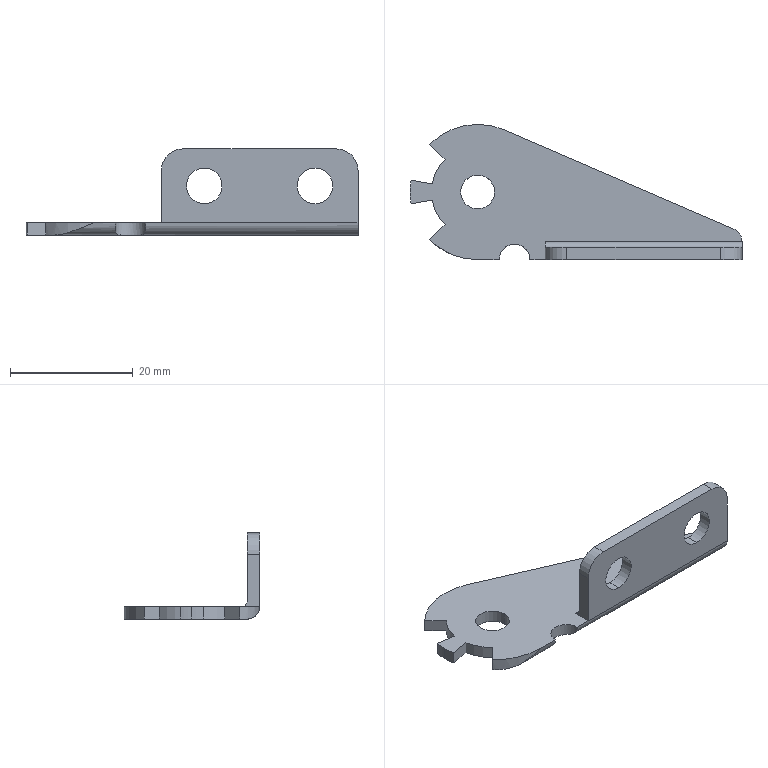Component | SolidWorks | MHPUS204-38-33-A-1_36-1 | 1 solid | 31 faces | box 54 x 22 x 14 mm | volume 2031 mm3 | cylinder 19 | plane 12 | commonest cylinder face diameters 22 x4 5.8 x4 5.5 x2 4 x2 15 x2 7 x2 5 x1 4.4 x1
STEP:
#1=COLOUR_RGB('',0.7922,0.8196,0.9333);
#2=FILL_AREA_STYLE_COLOUR('',#1);
#3=FILL_AREA_STYLE('',(#2));
#4=SURFACE_STYLE_FILL_AREA(#3);
#5=SURFACE_SIDE_STYLE('',(#4));
#6=SURFACE_STYLE_USAGE(.BOTH.,#5);
#7=PRESENTATION_STYLE_ASSIGNMENT((#6));
#8=CARTESIAN_POINT('',(0.1718,-3.898,2.047));
#9=VERTEX_POINT('',#8);
#10=CARTESIAN_POINT('',(-0.04475,-3.898,2.047));
#11=VERTEX_POINT('',#10);
#12=CARTESIAN_POINT('',(0.06352,-3.898,2.047));
#13=DIRECTION('',(0.,0.,-1.));
#14=DIRECTION('',(-1.,0.,0.));
#15=AXIS2_PLACEMENT_3D('',#12,#13,#14);
#16=CIRCLE('',#15,0.1083);
#17=EDGE_CURVE('',#9,#11,#16,.T.);
#18=ORIENTED_EDGE('',*,*,#17,.F.);
#19=CARTESIAN_POINT('',(0.1718,-3.898,1.969));
#20=VERTEX_POINT('',#19);
#21=CARTESIAN_POINT('',(0.1718,-3.898,1.969));
#22=DIRECTION('',(0.,0.,-1.));
#23=VECTOR('',#22,39.37);
#24=LINE('',#21,#23);
#25=EDGE_CURVE('',#9,#20,#24,.T.);
#26=ORIENTED_EDGE('',*,*,#25,.T.);
#27=CARTESIAN_POINT('',(-0.04475,-3.898,1.969));
#28=VERTEX_POINT('',#27);
#29=CARTESIAN_POINT('',(0.06352,-3.898,1.969));
#30=DIRECTION('',(0.,0.,-1.));
#31=DIRECTION('',(-1.,0.,0.));
#32=AXIS2_PLACEMENT_3D('',#29,#30,#31);
#33=CIRCLE('',#32,0.1083);
#34=EDGE_CURVE('',#20,#28,#33,.T.);
#35=ORIENTED_EDGE('',*,*,#34,.T.);
#36=CARTESIAN_POINT('',(-0.04475,-3.898,1.969));
#37=DIRECTION('',(0.,0.,-1.));
#38=VECTOR('',#37,39.37);
#39=LINE('',#36,#38);
#40=EDGE_CURVE('',#11,#28,#39,.T.);
#41=ORIENTED_EDGE('',*,*,#40,.F.);
#42=EDGE_LOOP('',(#18,#26,#35,#41));
#43=FACE_OUTER_BOUND('',#42,.T.);
#44=CARTESIAN_POINT('',(0.06352,-3.898,1.969));
#45=DIRECTION('',(0.,0.,-1.));
#46=DIRECTION('',(-1.,0.,0.));
#47=AXIS2_PLACEMENT_3D('',#44,#45,#46);
#48=CYLINDRICAL_SURFACE('',#47,0.1083);
#49=ADVANCED_FACE('',(#43),#48,.F.);
#50=CARTESIAN_POINT('',(-0.363,-3.973,2.047));
#51=VERTEX_POINT('',#50);
#52=CARTESIAN_POINT('',(-0.3696,-3.898,2.047));
#53=VERTEX_POINT('',#52);
#54=CARTESIAN_POINT('',(0.06352,-3.898,2.047));
#55=DIRECTION('',(0.,0.,-1.));
#56=DIRECTION('',(-1.,0.,0.));
#57=AXIS2_PLACEMENT_3D('',#54,#55,#56);
#58=CIRCLE('',#57,0.4331);
#59=EDGE_CURVE('',#51,#53,#58,.T.);
#60=ORIENTED_EDGE('',*,*,#59,.T.);
#61=CARTESIAN_POINT('',(-0.3696,-3.898,1.969));
#62=VERTEX_POINT('',#61);
#63=CARTESIAN_POINT('',(-0.3696,-3.898,1.969));
#64=DIRECTION('',(0.,0.,-1.));
#65=VECTOR('',#64,39.37);
#66=LINE('',#63,#65);
#67=EDGE_CURVE('',#53,#62,#66,.T.);
#68=ORIENTED_EDGE('',*,*,#67,.T.);
#69=CARTESIAN_POINT('',(-0.363,-3.973,1.969));
#70=VERTEX_POINT('',#69);
#71=CARTESIAN_POINT('',(0.06352,-3.898,1.969));
#72=DIRECTION('',(0.,0.,1.));
#73=DIRECTION('',(-1.,0.,0.));
#74=AXIS2_PLACEMENT_3D('',#71,#72,#73);
#75=CIRCLE('',#74,0.4331);
#76=EDGE_CURVE('',#62,#70,#75,.T.);
#77=ORIENTED_EDGE('',*,*,#76,.T.);
#78=CARTESIAN_POINT('',(-0.363,-3.973,1.969));
#79=DIRECTION('',(0.,0.,-1.));
#80=VECTOR('',#79,39.37);
#81=LINE('',#78,#80);
#82=EDGE_CURVE('',#51,#70,#81,.T.);
#83=ORIENTED_EDGE('',*,*,#82,.F.);
#84=EDGE_LOOP('',(#60,#68,#77,#83));
#85=FACE_OUTER_BOUND('',#84,.T.);
#86=CARTESIAN_POINT('',(0.06352,-3.898,1.969));
#87=DIRECTION('',(0.,0.,-1.));
#88=DIRECTION('',(-1.,0.,0.));
#89=AXIS2_PLACEMENT_3D('',#86,#87,#88);
#90=CYLINDRICAL_SURFACE('',#89,0.4331);
#91=ADVANCED_FACE('',(#85),#90,.T.);
#92=CARTESIAN_POINT('',(0.7722,-4.252,2.169));
#93=VERTEX_POINT('',#92);
#94=CARTESIAN_POINT('',(0.7722,-4.252,2.398));
#95=VERTEX_POINT('',#94);
#96=CARTESIAN_POINT('',(0.7722,-4.252,2.283));
#97=DIRECTION('',(0.,1.,0.));
#98=DIRECTION('',(0.,0.,-1.));
#99=AXIS2_PLACEMENT_3D('',#96,#97,#98);
#100=CIRCLE('',#99,0.1142);
#101=EDGE_CURVE('',#93,#95,#100,.T.);
#102=ORIENTED_EDGE('',*,*,#101,.T.);
#103=CARTESIAN_POINT('',(0.7722,-4.331,2.398));
#104=VERTEX_POINT('',#103);
#105=CARTESIAN_POINT('',(0.7722,-4.331,2.398));
#106=DIRECTION('',(0.,-1.,0.));
#107=VECTOR('',#106,39.37);
#108=LINE('',#105,#107);
#109=EDGE_CURVE('',#95,#104,#108,.T.);
#110=ORIENTED_EDGE('',*,*,#109,.T.);
#111=CARTESIAN_POINT('',(0.7722,-4.331,2.169));
#112=VERTEX_POINT('',#111);
#113=CARTESIAN_POINT('',(0.7722,-4.331,2.283));
#114=DIRECTION('',(0.,1.,0.));
#115=DIRECTION('',(0.,0.,-1.));
#116=AXIS2_PLACEMENT_3D('',#113,#114,#115);
#117=CIRCLE('',#116,0.1142);
#118=EDGE_CURVE('',#112,#104,#117,.T.);
#119=ORIENTED_EDGE('',*,*,#118,.F.);
#120=CARTESIAN_POINT('',(0.7722,-4.331,2.169));
#121=DIRECTION('',(0.,-1.,0.));
#122=VECTOR('',#121,39.37);
#123=LINE('',#120,#122);
#124=EDGE_CURVE('',#93,#112,#123,.T.);
#125=ORIENTED_EDGE('',*,*,#124,.F.);
#126=EDGE_LOOP('',(#102,#110,#119,#125));
#127=FACE_OUTER_BOUND('',#126,.T.);
#128=CARTESIAN_POINT('',(0.7722,-4.331,2.283));
#129=DIRECTION('',(0.,-1.,0.));
#130=DIRECTION('',(0.,0.,-1.));
#131=AXIS2_PLACEMENT_3D('',#128,#129,#130);
#132=CYLINDRICAL_SURFACE('',#131,0.1142);
#133=ADVANCED_FACE('',(#127),#132,.F.);
#134=CARTESIAN_POINT('',(1.481,-4.252,2.169));
#135=VERTEX_POINT('',#134);
#136=CARTESIAN_POINT('',(1.481,-4.252,2.398));
#137=VERTEX_POINT('',#136);
#138=CARTESIAN_POINT('',(1.481,-4.252,2.283));
#139=DIRECTION('',(0.,1.,0.));
#140=DIRECTION('',(0.,0.,-1.));
#141=AXIS2_PLACEMENT_3D('',#138,#139,#140);
#142=CIRCLE('',#141,0.1142);
#143=EDGE_CURVE('',#135,#137,#142,.T.);
#144=ORIENTED_EDGE('',*,*,#143,.T.);
#145=CARTESIAN_POINT('',(1.481,-4.331,2.398));
#146=VERTEX_POINT('',#145);
#147=CARTESIAN_POINT('',(1.481,-4.331,2.398));
#148=DIRECTION('',(0.,-1.,0.));
#149=VECTOR('',#148,39.37);
#150=LINE('',#147,#149);
#151=EDGE_CURVE('',#137,#146,#150,.T.);
#152=ORIENTED_EDGE('',*,*,#151,.T.);
#153=CARTESIAN_POINT('',(1.481,-4.331,2.169));
#154=VERTEX_POINT('',#153);
#155=CARTESIAN_POINT('',(1.481,-4.331,2.283));
#156=DIRECTION('',(0.,1.,0.));
#157=DIRECTION('',(0.,0.,-1.));
#158=AXIS2_PLACEMENT_3D('',#155,#156,#157);
#159=CIRCLE('',#158,0.1142);
#160=EDGE_CURVE('',#154,#146,#159,.T.);
#161=ORIENTED_EDGE('',*,*,#160,.F.);
#162=CARTESIAN_POINT('',(1.481,-4.331,2.169));
#163=DIRECTION('',(0.,-1.,0.));
#164=VECTOR('',#163,39.37);
#165=LINE('',#162,#164);
#166=EDGE_CURVE('',#135,#154,#165,.T.);
#167=ORIENTED_EDGE('',*,*,#166,.F.);
#168=EDGE_LOOP('',(#144,#152,#161,#167));
#169=FACE_OUTER_BOUND('',#168,.T.);
#170=CARTESIAN_POINT('',(1.481,-4.331,2.283));
#171=DIRECTION('',(0.,-1.,0.));
#172=DIRECTION('',(0.,0.,-1.));
#173=AXIS2_PLACEMENT_3D('',#170,#171,#172);
#174=CYLINDRICAL_SURFACE('',#173,0.1142);
#175=ADVANCED_FACE('',(#169),#174,.F.);
#176=CARTESIAN_POINT('',(0.06352,-3.898,1.969));
#177=DIRECTION('',(0.,0.,-1.));
#178=DIRECTION('',(-1.,0.,0.));
#179=AXIS2_PLACEMENT_3D('',#176,#177,#178);
#180=CIRCLE('',#179,0.1083);
#181=EDGE_CURVE('',#28,#20,#180,.T.);
#182=ORIENTED_EDGE('',*,*,#181,.F.);
#183=ORIENTED_EDGE('',*,*,#34,.F.);
#184=EDGE_LOOP('',(#182,#183));
#185=FACE_BOUND('',#184,.T.);
#186=CARTESIAN_POINT('',(-0.1855,-4.252,1.969));
#187=VERTEX_POINT('',#186);
#188=CARTESIAN_POINT('',(0.2407,-4.252,1.969));
#189=VERTEX_POINT('',#188);
#190=CARTESIAN_POINT('',(0.06352,-4.252,1.969));
#191=DIRECTION('',(1.,0.,0.));
#192=VECTOR('',#191,39.37);
#193=LINE('',#190,#192);
#194=EDGE_CURVE('',#187,#189,#193,.T.);
#195=ORIENTED_EDGE('',*,*,#194,.F.);
#196=CARTESIAN_POINT('',(-0.2427,-4.204,1.969));
#197=VERTEX_POINT('',#196);
#198=CARTESIAN_POINT('',(0.06352,-3.898,1.969));
#199=DIRECTION('',(0.,0.,1.));
#200=DIRECTION('',(-1.,-0.,0.));
#201=AXIS2_PLACEMENT_3D('',#198,#199,#200);
#202=CIRCLE('',#201,0.4331);
#203=EDGE_CURVE('',#197,#187,#202,.T.);
#204=ORIENTED_EDGE('',*,*,#203,.F.);
#205=CARTESIAN_POINT('',(-0.1453,-4.106,1.969));
#206=VERTEX_POINT('',#205);
#207=CARTESIAN_POINT('',(-0.1453,-4.106,1.969));
#208=DIRECTION('',(-0.7071,-0.7071,0.));
#209=VECTOR('',#208,39.37);
#210=LINE('',#207,#209);
#211=EDGE_CURVE('',#206,#197,#210,.T.);
#212=ORIENTED_EDGE('',*,*,#211,.F.);
#213=CARTESIAN_POINT('',(-0.2273,-3.949,1.969));
#214=VERTEX_POINT('',#213);
#215=CARTESIAN_POINT('',(0.06352,-3.898,1.969));
#216=DIRECTION('',(0.,0.,1.));
#217=DIRECTION('',(-1.,0.,0.));
#218=AXIS2_PLACEMENT_3D('',#215,#216,#217);
#219=CIRCLE('',#218,0.2953);
#220=EDGE_CURVE('',#214,#206,#219,.T.);
#221=ORIENTED_EDGE('',*,*,#220,.F.);
#222=CARTESIAN_POINT('',(-0.363,-3.973,1.969));
#223=DIRECTION('',(0.9848,0.1736,0.));
#224=VECTOR('',#223,39.37);
#225=LINE('',#222,#224);
#226=EDGE_CURVE('',#70,#214,#225,.T.);
#227=ORIENTED_EDGE('',*,*,#226,.F.);
#228=ORIENTED_EDGE('',*,*,#76,.F.);
#229=CARTESIAN_POINT('',(-0.363,-3.822,1.969));
#230=VERTEX_POINT('',#229);
#231=CARTESIAN_POINT('',(0.06352,-3.898,1.969));
#232=DIRECTION('',(0.,0.,1.));
#233=DIRECTION('',(-1.,0.,0.));
#234=AXIS2_PLACEMENT_3D('',#231,#232,#233);
#235=CIRCLE('',#234,0.4331);
#236=EDGE_CURVE('',#230,#62,#235,.T.);
#237=ORIENTED_EDGE('',*,*,#236,.F.);
#238=CARTESIAN_POINT('',(-0.2273,-3.846,1.969));
#239=VERTEX_POINT('',#238);
#240=CARTESIAN_POINT('',(-0.2273,-3.846,1.969));
#241=DIRECTION('',(-0.9848,0.1736,0.));
#242=VECTOR('',#241,39.37);
#243=LINE('',#240,#242);
#244=EDGE_CURVE('',#239,#230,#243,.T.);
#245=ORIENTED_EDGE('',*,*,#244,.F.);
#246=CARTESIAN_POINT('',(-0.1453,-3.689,1.969));
#247=VERTEX_POINT('',#246);
#248=CARTESIAN_POINT('',(0.06352,-3.898,1.969));
#249=DIRECTION('',(0.,0.,1.));
#250=DIRECTION('',(-1.,0.,0.));
#251=AXIS2_PLACEMENT_3D('',#248,#249,#250);
#252=CIRCLE('',#251,0.2953);
#253=EDGE_CURVE('',#247,#239,#252,.T.);
#254=ORIENTED_EDGE('',*,*,#253,.F.);
#255=CARTESIAN_POINT('',(-0.2427,-3.591,1.969));
#256=VERTEX_POINT('',#255);
#257=CARTESIAN_POINT('',(-0.2427,-3.591,1.969));
#258=DIRECTION('',(0.7071,-0.7071,0.));
#259=VECTOR('',#258,39.37);
#260=LINE('',#257,#259);
#261=EDGE_CURVE('',#256,#247,#260,.T.);
#262=ORIENTED_EDGE('',*,*,#261,.F.);
#263=CARTESIAN_POINT('',(0.2353,-3.5,1.969));
#264=VERTEX_POINT('',#263);
#265=CARTESIAN_POINT('',(0.06352,-3.898,1.969));
#266=DIRECTION('',(0.,0.,1.));
#267=DIRECTION('',(-1.,-0.,0.));
#268=AXIS2_PLACEMENT_3D('',#265,#266,#267);
#269=CIRCLE('',#268,0.4331);
#270=EDGE_CURVE('',#264,#256,#269,.T.);
#271=ORIENTED_EDGE('',*,*,#270,.F.);
#272=CARTESIAN_POINT('',(1.704,-4.135,1.969));
#273=VERTEX_POINT('',#272);
#274=CARTESIAN_POINT('',(1.704,-4.135,1.969));
#275=DIRECTION('',(-0.9179,0.3967,0.));
#276=VECTOR('',#275,39.37);
#277=LINE('',#274,#276);
#278=EDGE_CURVE('',#273,#264,#277,.T.);
#279=ORIENTED_EDGE('',*,*,#278,.F.);
#280=CARTESIAN_POINT('',(1.756,-4.214,1.969));
#281=VERTEX_POINT('',#280);
#282=CARTESIAN_POINT('',(1.67,-4.214,1.969));
#283=DIRECTION('',(0.,0.,1.));
#284=DIRECTION('',(-1.,-0.,0.));
#285=AXIS2_PLACEMENT_3D('',#282,#283,#284);
#286=CIRCLE('',#285,0.08661);
#287=EDGE_CURVE('',#281,#273,#286,.T.);
#288=ORIENTED_EDGE('',*,*,#287,.F.);
#289=CARTESIAN_POINT('',(1.756,-4.252,1.969));
#290=VERTEX_POINT('',#289);
#291=CARTESIAN_POINT('',(1.756,-4.214,1.969));
#292=DIRECTION('',(0.,1.,0.));
#293=VECTOR('',#292,39.37);
#294=LINE('',#291,#293);
#295=EDGE_CURVE('',#290,#281,#294,.T.);
#296=ORIENTED_EDGE('',*,*,#295,.F.);
#297=CARTESIAN_POINT('',(0.3588,-4.252,1.969));
#298=VERTEX_POINT('',#297);
#299=CARTESIAN_POINT('',(0.06352,-4.252,1.969));
#300=DIRECTION('',(1.,0.,0.));
#301=VECTOR('',#300,39.37);
#302=LINE('',#299,#301);
#303=EDGE_CURVE('',#298,#290,#302,.T.);
#304=ORIENTED_EDGE('',*,*,#303,.F.);
#305=CARTESIAN_POINT('',(0.2997,-4.331,1.969));
#306=DIRECTION('',(0.,0.,-1.));
#307=DIRECTION('',(-1.,0.,0.));
#308=AXIS2_PLACEMENT_3D('',#305,#306,#307);
#309=CIRCLE('',#308,0.09843);
#310=EDGE_CURVE('',#189,#298,#309,.T.);
#311=ORIENTED_EDGE('',*,*,#310,.F.);
#312=EDGE_LOOP('',(#195,#204,#212,#221,#227,#228,#237,#245,#254,#262,#271,#279,#288,#296,#304,#311));
#313=FACE_OUTER_BOUND('',#312,.T.);
#314=CARTESIAN_POINT('',(0.06352,-4.331,1.969));
#315=DIRECTION('',(0.,0.,1.));
#316=DIRECTION('',(1.,0.,0.));
#317=AXIS2_PLACEMENT_3D('',#314,#315,#316);
#318=PLANE('',#317);
#319=ADVANCED_FACE('',(#185,#313),#318,.F.);
#320=ORIENTED_EDGE('',*,*,#25,.F.);
#321=CARTESIAN_POINT('',(0.06352,-3.898,2.047));
#322=DIRECTION('',(0.,0.,-1.));
#323=DIRECTION('',(-1.,0.,0.));
#324=AXIS2_PLACEMENT_3D('',#321,#322,#323);
#325=CIRCLE('',#324,0.1083);
#326=EDGE_CURVE('',#11,#9,#325,.T.);
#327=ORIENTED_EDGE('',*,*,#326,.F.);
#328=ORIENTED_EDGE('',*,*,#40,.T.);
#329=ORIENTED_EDGE('',*,*,#181,.T.);
#330=EDGE_LOOP('',(#320,#327,#328,#329));
#331=FACE_OUTER_BOUND('',#330,.T.);
#332=CARTESIAN_POINT('',(0.06352,-3.898,1.969));
#333=DIRECTION('',(0.,0.,-1.));
#334=DIRECTION('',(-1.,0.,0.));
#335=AXIS2_PLACEMENT_3D('',#332,#333,#334);
#336=CYLINDRICAL_SURFACE('',#335,0.1083);
#337=ADVANCED_FACE('',(#331),#336,.F.);
#338=CARTESIAN_POINT('',(0.2013,-4.331,2.047));
#339=VERTEX_POINT('',#338);
#340=CARTESIAN_POINT('',(0.3982,-4.331,2.047));
#341=VERTEX_POINT('',#340);
#342=CARTESIAN_POINT('',(0.2997,-4.331,2.047));
#343=DIRECTION('',(0.,0.,-1.));
#344=DIRECTION('',(-1.,0.,0.));
#345=AXIS2_PLACEMENT_3D('',#342,#343,#344);
#346=CIRCLE('',#345,0.09843);
#347=EDGE_CURVE('',#339,#341,#346,.T.);
#348=ORIENTED_EDGE('',*,*,#347,.F.);
#349=CARTESIAN_POINT('',(0.2407,-4.252,1.969));
#350=CARTESIAN_POINT('',(0.2361,-4.255,1.969));
#351=CARTESIAN_POINT('',(0.2319,-4.259,1.969));
#352=CARTESIAN_POINT('',(0.2243,-4.267,1.97));
#353=CARTESIAN_POINT('',(0.2207,-4.272,1.971));
#354=CARTESIAN_POINT('',(0.2147,-4.281,1.974));
#355=CARTESIAN_POINT('',(0.2122,-4.285,1.976));
#356=CARTESIAN_POINT('',(0.208,-4.295,1.981));
#357=CARTESIAN_POINT('',(0.2064,-4.299,1.984));
#358=CARTESIAN_POINT('',(0.204,-4.307,1.991));
#359=CARTESIAN_POINT('',(0.2032,-4.311,1.995));
#360=CARTESIAN_POINT('',(0.2021,-4.318,2.004));
#361=CARTESIAN_POINT('',(0.2018,-4.321,2.009));
#362=CARTESIAN_POINT('',(0.2014,-4.326,2.019));
#363=CARTESIAN_POINT('',(0.2014,-4.328,2.025));
#364=CARTESIAN_POINT('',(0.2013,-4.33,2.036));
#365=CARTESIAN_POINT('',(0.2013,-4.331,2.042));
#366=CARTESIAN_POINT('',(0.2013,-4.331,2.047));
#367=B_SPLINE_CURVE_WITH_KNOTS('',3,(#349,#350,#351,#352,#353,#354,#355,#356,#357,#358,#359,#360,#361,#362,#363,#364,#365,#366),.UNSPECIFIED.,.F.,.F.,(4,2,2,2,2,2,2,2,4),(0.,0.0004287,0.0008574,0.001286,0.001715,0.002144,0.002572,0.003001,0.00343),.UNSPECIFIED.);
#368=EDGE_CURVE('',#189,#339,#367,.T.);
#369=ORIENTED_EDGE('',*,*,#368,.F.);
#370=ORIENTED_EDGE('',*,*,#310,.T.);
#371=CARTESIAN_POINT('',(0.3982,-4.331,2.047));
#372=CARTESIAN_POINT('',(0.3982,-4.331,2.042));
#373=CARTESIAN_POINT('',(0.3982,-4.33,2.036));
#374=CARTESIAN_POINT('',(0.3981,-4.328,2.025));
#375=CARTESIAN_POINT('',(0.3981,-4.326,2.019));
#376=CARTESIAN_POINT('',(0.3977,-4.321,2.009));
#377=CARTESIAN_POINT('',(0.3974,-4.318,2.004));
#378=CARTESIAN_POINT('',(0.3963,-4.311,1.995));
#379=CARTESIAN_POINT('',(0.3955,-4.308,1.991));
#380=CARTESIAN_POINT('',(0.3931,-4.299,1.984));
#381=CARTESIAN_POINT('',(0.3915,-4.295,1.981));
#382=CARTESIAN_POINT('',(0.3874,-4.286,1.976));
#383=CARTESIAN_POINT('',(0.3849,-4.281,1.974));
#384=CARTESIAN_POINT('',(0.3757,-4.267,1.969));
#385=CARTESIAN_POINT('',(0.3679,-4.259,1.969));
#386=CARTESIAN_POINT('',(0.3588,-4.252,1.969));
#387=B_SPLINE_CURVE_WITH_KNOTS('',3,(#371,#372,#373,#374,#375,#376,#377,#378,#379,#380,#381,#382,#383,#384,#385,#386),.UNSPECIFIED.,.F.,.F.,(4,2,2,2,2,2,2,4),(0.,0.0004284,0.0008569,0.001285,0.001714,0.002142,0.002571,0.003428),.UNSPECIFIED.);
#388=EDGE_CURVE('',#341,#298,#387,.T.);
#389=ORIENTED_EDGE('',*,*,#388,.F.);
#390=EDGE_LOOP('',(#348,#369,#370,#389));
#391=FACE_OUTER_BOUND('',#390,.T.);
#392=CARTESIAN_POINT('',(0.2997,-4.331,1.969));
#393=DIRECTION('',(0.,0.,-1.));
#394=DIRECTION('',(-1.,0.,0.));
#395=AXIS2_PLACEMENT_3D('',#392,#393,#394);
#396=CYLINDRICAL_SURFACE('',#395,0.09843);
#397=ADVANCED_FACE('',(#391),#396,.F.);
#398=CARTESIAN_POINT('',(0.06352,-4.331,2.047));
#399=VERTEX_POINT('',#398);
#400=CARTESIAN_POINT('',(0.06352,-4.331,2.047));
#401=CARTESIAN_POINT('',(0.04212,-4.331,2.038));
#402=CARTESIAN_POINT('',(0.02068,-4.329,2.029));
#403=CARTESIAN_POINT('',(-0.02198,-4.323,2.011));
#404=CARTESIAN_POINT('',(-0.04301,-4.318,2.003));
#405=CARTESIAN_POINT('',(-0.0743,-4.308,1.992));
#406=CARTESIAN_POINT('',(-0.08469,-4.305,1.989));
#407=CARTESIAN_POINT('',(-0.1054,-4.297,1.982));
#408=CARTESIAN_POINT('',(-0.1158,-4.292,1.979));
#409=CARTESIAN_POINT('',(-0.1465,-4.277,1.972));
#410=CARTESIAN_POINT('',(-0.1663,-4.265,1.969));
#411=CARTESIAN_POINT('',(-0.1855,-4.252,1.969));
#412=B_SPLINE_CURVE_WITH_KNOTS('',3,(#400,#401,#402,#403,#404,#405,#406,#407,#408,#409,#410,#411),.UNSPECIFIED.,.F.,.F.,(4,2,2,2,2,4),(-0.00002098,0.001752,0.003524,0.004411,0.005297,0.00707),.UNSPECIFIED.);
#413=EDGE_CURVE('',#399,#187,#412,.T.);
#414=ORIENTED_EDGE('',*,*,#413,.T.);
#415=ORIENTED_EDGE('',*,*,#194,.T.);
#416=ORIENTED_EDGE('',*,*,#368,.T.);
#417=CARTESIAN_POINT('',(1.756,-4.331,2.047));
#418=DIRECTION('',(-1.,0.,0.));
#419=VECTOR('',#418,39.37);
#420=LINE('',#417,#419);
#421=EDGE_CURVE('',#339,#399,#420,.T.);
#422=ORIENTED_EDGE('',*,*,#421,.T.);
#423=EDGE_LOOP('',(#414,#415,#416,#422));
#424=FACE_OUTER_BOUND('',#423,.T.);
#425=CARTESIAN_POINT('',(1.756,-4.252,2.047));
#426=DIRECTION('',(1.,0.,0.));
#427=DIRECTION('',(0.,0.,-1.));
#428=AXIS2_PLACEMENT_3D('',#425,#426,#427);
#429=CYLINDRICAL_SURFACE('',#428,0.07874);
#430=ADVANCED_FACE('',(#424),#429,.T.);
#431=ORIENTED_EDGE('',*,*,#203,.T.);
#432=ORIENTED_EDGE('',*,*,#413,.F.);
#433=CARTESIAN_POINT('',(-0.2427,-4.204,2.047));
#434=VERTEX_POINT('',#433);
#435=CARTESIAN_POINT('',(0.06352,-3.898,2.047));
#436=DIRECTION('',(0.,0.,-1.));
#437=DIRECTION('',(-1.,0.,0.));
#438=AXIS2_PLACEMENT_3D('',#435,#436,#437);
#439=CIRCLE('',#438,0.4331);
#440=EDGE_CURVE('',#399,#434,#439,.T.);
#441=ORIENTED_EDGE('',*,*,#440,.T.);
#442=CARTESIAN_POINT('',(-0.2427,-4.204,1.969));
#443=DIRECTION('',(0.,0.,-1.));
#444=VECTOR('',#443,39.37);
#445=LINE('',#442,#444);
#446=EDGE_CURVE('',#434,#197,#445,.T.);
#447=ORIENTED_EDGE('',*,*,#446,.T.);
#448=EDGE_LOOP('',(#431,#432,#441,#447));
#449=FACE_OUTER_BOUND('',#448,.T.);
#450=CARTESIAN_POINT('',(0.06352,-3.898,1.969));
#451=DIRECTION('',(0.,0.,-1.));
#452=DIRECTION('',(-1.,0.,0.));
#453=AXIS2_PLACEMENT_3D('',#450,#451,#452);
#454=CYLINDRICAL_SURFACE('',#453,0.4331);
#455=ADVANCED_FACE('',(#449),#454,.T.);
#456=ORIENTED_EDGE('',*,*,#211,.T.);
#457=ORIENTED_EDGE('',*,*,#446,.F.);
#458=CARTESIAN_POINT('',(-0.1453,-4.106,2.047));
#459=VERTEX_POINT('',#458);
#460=CARTESIAN_POINT('',(-0.2427,-4.204,2.047));
#461=DIRECTION('',(0.7071,0.7071,0.));
#462=VECTOR('',#461,39.37);
#463=LINE('',#460,#462);
#464=EDGE_CURVE('',#434,#459,#463,.T.);
#465=ORIENTED_EDGE('',*,*,#464,.T.);
#466=CARTESIAN_POINT('',(-0.1453,-4.106,1.969));
#467=DIRECTION('',(0.,0.,-1.));
#468=VECTOR('',#467,39.37);
#469=LINE('',#466,#468);
#470=EDGE_CURVE('',#459,#206,#469,.T.);
#471=ORIENTED_EDGE('',*,*,#470,.T.);
#472=EDGE_LOOP('',(#456,#457,#465,#471));
#473=FACE_OUTER_BOUND('',#472,.T.);
#474=CARTESIAN_POINT('',(-0.2427,-4.204,1.969));
#475=DIRECTION('',(-0.7071,0.7071,0.));
#476=DIRECTION('',(-0.7071,-0.7071,0.));
#477=AXIS2_PLACEMENT_3D('',#474,#475,#476);
#478=PLANE('',#477);
#479=ADVANCED_FACE('',(#473),#478,.T.);
#480=ORIENTED_EDGE('',*,*,#220,.T.);
#481=ORIENTED_EDGE('',*,*,#470,.F.);
#482=CARTESIAN_POINT('',(-0.2273,-3.949,2.047));
#483=VERTEX_POINT('',#482);
#484=CARTESIAN_POINT('',(0.06352,-3.898,2.047));
#485=DIRECTION('',(0.,0.,-1.));
#486=DIRECTION('',(-1.,0.,0.));
#487=AXIS2_PLACEMENT_3D('',#484,#485,#486);
#488=CIRCLE('',#487,0.2953);
#489=EDGE_CURVE('',#459,#483,#488,.T.);
#490=ORIENTED_EDGE('',*,*,#489,.T.);
#491=CARTESIAN_POINT('',(-0.2273,-3.949,1.969));
#492=DIRECTION('',(0.,0.,-1.));
#493=VECTOR('',#492,39.37);
#494=LINE('',#491,#493);
#495=EDGE_CURVE('',#483,#214,#494,.T.);
#496=ORIENTED_EDGE('',*,*,#495,.T.);
#497=EDGE_LOOP('',(#480,#481,#490,#496));
#498=FACE_OUTER_BOUND('',#497,.T.);
#499=CARTESIAN_POINT('',(0.06352,-3.898,1.969));
#500=DIRECTION('',(0.,0.,-1.));
#501=DIRECTION('',(-1.,0.,0.));
#502=AXIS2_PLACEMENT_3D('',#499,#500,#501);
#503=CYLINDRICAL_SURFACE('',#502,0.2953);
#504=ADVANCED_FACE('',(#498),#503,.T.);
#505=ORIENTED_EDGE('',*,*,#226,.T.);
#506=ORIENTED_EDGE('',*,*,#495,.F.);
#507=CARTESIAN_POINT('',(-0.2273,-3.949,2.047));
#508=DIRECTION('',(-0.9848,-0.1736,0.));
#509=VECTOR('',#508,39.37);
#510=LINE('',#507,#509);
#511=EDGE_CURVE('',#483,#51,#510,.T.);
#512=ORIENTED_EDGE('',*,*,#511,.T.);
#513=ORIENTED_EDGE('',*,*,#82,.T.);
#514=EDGE_LOOP('',(#505,#506,#512,#513));
#515=FACE_OUTER_BOUND('',#514,.T.);
#516=CARTESIAN_POINT('',(-0.2273,-3.949,1.969));
#517=DIRECTION('',(0.1736,-0.9848,0.));
#518=DIRECTION('',(0.9848,0.1736,0.));
#519=AXIS2_PLACEMENT_3D('',#516,#517,#518);
#520=PLANE('',#519);
#521=ADVANCED_FACE('',(#515),#520,.T.);
#522=ORIENTED_EDGE('',*,*,#67,.F.);
#523=CARTESIAN_POINT('',(-0.363,-3.822,2.047));
#524=VERTEX_POINT('',#523);
#525=CARTESIAN_POINT('',(0.06352,-3.898,2.047));
#526=DIRECTION('',(0.,0.,-1.));
#527=DIRECTION('',(-1.,0.,0.));
#528=AXIS2_PLACEMENT_3D('',#525,#526,#527);
#529=CIRCLE('',#528,0.4331);
#530=EDGE_CURVE('',#53,#524,#529,.T.);
#531=ORIENTED_EDGE('',*,*,#530,.T.);
#532=CARTESIAN_POINT('',(-0.363,-3.822,1.969));
#533=DIRECTION('',(0.,0.,-1.));
#534=VECTOR('',#533,39.37);
#535=LINE('',#532,#534);
#536=EDGE_CURVE('',#524,#230,#535,.T.);
#537=ORIENTED_EDGE('',*,*,#536,.T.);
#538=ORIENTED_EDGE('',*,*,#236,.T.);
#539=EDGE_LOOP('',(#522,#531,#537,#538));
#540=FACE_OUTER_BOUND('',#539,.T.);
#541=CARTESIAN_POINT('',(0.06352,-3.898,1.969));
#542=DIRECTION('',(0.,0.,-1.));
#543=DIRECTION('',(-1.,0.,0.));
#544=AXIS2_PLACEMENT_3D('',#541,#542,#543);
#545=CYLINDRICAL_SURFACE('',#544,0.4331);
#546=ADVANCED_FACE('',(#540),#545,.T.);
#547=ORIENTED_EDGE('',*,*,#244,.T.);
#548=ORIENTED_EDGE('',*,*,#536,.F.);
#549=CARTESIAN_POINT('',(-0.2273,-3.846,2.047));
#550=VERTEX_POINT('',#549);
#551=CARTESIAN_POINT('',(-0.363,-3.822,2.047));
#552=DIRECTION('',(0.9848,-0.1736,0.));
#553=VECTOR('',#552,39.37);
#554=LINE('',#551,#553);
#555=EDGE_CURVE('',#524,#550,#554,.T.);
#556=ORIENTED_EDGE('',*,*,#555,.T.);
#557=CARTESIAN_POINT('',(-0.2273,-3.846,1.969));
#558=DIRECTION('',(0.,0.,-1.));
#559=VECTOR('',#558,39.37);
#560=LINE('',#557,#559);
#561=EDGE_CURVE('',#550,#239,#560,.T.);
#562=ORIENTED_EDGE('',*,*,#561,.T.);
#563=EDGE_LOOP('',(#547,#548,#556,#562));
#564=FACE_OUTER_BOUND('',#563,.T.);
#565=CARTESIAN_POINT('',(-0.363,-3.822,1.969));
#566=DIRECTION('',(0.1736,0.9848,0.));
#567=DIRECTION('',(-0.9848,0.1736,0.));
#568=AXIS2_PLACEMENT_3D('',#565,#566,#567);
#569=PLANE('',#568);
#570=ADVANCED_FACE('',(#564),#569,.T.);
#571=ORIENTED_EDGE('',*,*,#253,.T.);
#572=ORIENTED_EDGE('',*,*,#561,.F.);
#573=CARTESIAN_POINT('',(-0.1453,-3.689,2.047));
#574=VERTEX_POINT('',#573);
#575=CARTESIAN_POINT('',(0.06352,-3.898,2.047));
#576=DIRECTION('',(0.,0.,-1.));
#577=DIRECTION('',(-1.,0.,0.));
#578=AXIS2_PLACEMENT_3D('',#575,#576,#577);
#579=CIRCLE('',#578,0.2953);
#580=EDGE_CURVE('',#550,#574,#579,.T.);
#581=ORIENTED_EDGE('',*,*,#580,.T.);
#582=CARTESIAN_POINT('',(-0.1453,-3.689,1.969));
#583=DIRECTION('',(0.,0.,-1.));
#584=VECTOR('',#583,39.37);
#585=LINE('',#582,#584);
#586=EDGE_CURVE('',#574,#247,#585,.T.);
#587=ORIENTED_EDGE('',*,*,#586,.T.);
#588=EDGE_LOOP('',(#571,#572,#581,#587));
#589=FACE_OUTER_BOUND('',#588,.T.);
#590=CARTESIAN_POINT('',(0.06352,-3.898,1.969));
#591=DIRECTION('',(0.,0.,-1.));
#592=DIRECTION('',(-1.,0.,0.));
#593=AXIS2_PLACEMENT_3D('',#590,#591,#592);
#594=CYLINDRICAL_SURFACE('',#593,0.2953);
#595=ADVANCED_FACE('',(#589),#594,.T.);
#596=ORIENTED_EDGE('',*,*,#261,.T.);
#597=ORIENTED_EDGE('',*,*,#586,.F.);
#598=CARTESIAN_POINT('',(-0.2427,-3.591,2.047));
#599=VERTEX_POINT('',#598);
#600=CARTESIAN_POINT('',(-0.1453,-3.689,2.047));
#601=DIRECTION('',(-0.7071,0.7071,0.));
#602=VECTOR('',#601,39.37);
#603=LINE('',#600,#602);
#604=EDGE_CURVE('',#574,#599,#603,.T.);
#605=ORIENTED_EDGE('',*,*,#604,.T.);
#606=CARTESIAN_POINT('',(-0.2427,-3.591,1.969));
#607=DIRECTION('',(0.,0.,-1.));
#608=VECTOR('',#607,39.37);
#609=LINE('',#606,#608);
#610=EDGE_CURVE('',#599,#256,#609,.T.);
#611=ORIENTED_EDGE('',*,*,#610,.T.);
#612=EDGE_LOOP('',(#596,#597,#605,#611));
#613=FACE_OUTER_BOUND('',#612,.T.);
#614=CARTESIAN_POINT('',(-0.1453,-3.689,1.969));
#615=DIRECTION('',(-0.7071,-0.7071,0.));
#616=DIRECTION('',(0.7071,-0.7071,0.));
#617=AXIS2_PLACEMENT_3D('',#614,#615,#616);
#618=PLANE('',#617);
#619=ADVANCED_FACE('',(#613),#618,.T.);
#620=ORIENTED_EDGE('',*,*,#270,.T.);
#621=ORIENTED_EDGE('',*,*,#610,.F.);
#622=CARTESIAN_POINT('',(0.2353,-3.5,2.047));
#623=VERTEX_POINT('',#622);
#624=CARTESIAN_POINT('',(0.06352,-3.898,2.047));
#625=DIRECTION('',(0.,0.,-1.));
#626=DIRECTION('',(-1.,0.,0.));
#627=AXIS2_PLACEMENT_3D('',#624,#625,#626);
#628=CIRCLE('',#627,0.4331);
#629=EDGE_CURVE('',#599,#623,#628,.T.);
#630=ORIENTED_EDGE('',*,*,#629,.T.);
#631=CARTESIAN_POINT('',(0.2353,-3.5,1.969));
#632=DIRECTION('',(0.,0.,-1.));
#633=VECTOR('',#632,39.37);
#634=LINE('',#631,#633);
#635=EDGE_CURVE('',#623,#264,#634,.T.);
#636=ORIENTED_EDGE('',*,*,#635,.T.);
#637=EDGE_LOOP('',(#620,#621,#630,#636));
#638=FACE_OUTER_BOUND('',#637,.T.);
#639=CARTESIAN_POINT('',(0.06352,-3.898,1.969));
#640=DIRECTION('',(0.,0.,-1.));
#641=DIRECTION('',(-1.,0.,0.));
#642=AXIS2_PLACEMENT_3D('',#639,#640,#641);
#643=CYLINDRICAL_SURFACE('',#642,0.4331);
#644=ADVANCED_FACE('',(#638),#643,.T.);
#645=ORIENTED_EDGE('',*,*,#278,.T.);
#646=ORIENTED_EDGE('',*,*,#635,.F.);
#647=CARTESIAN_POINT('',(1.704,-4.135,2.047));
#648=VERTEX_POINT('',#647);
#649=CARTESIAN_POINT('',(0.2353,-3.5,2.047));
#650=DIRECTION('',(0.9179,-0.3967,0.));
#651=VECTOR('',#650,39.37);
#652=LINE('',#649,#651);
#653=EDGE_CURVE('',#623,#648,#652,.T.);
#654=ORIENTED_EDGE('',*,*,#653,.T.);
#655=CARTESIAN_POINT('',(1.704,-4.135,1.969));
#656=DIRECTION('',(0.,0.,-1.));
#657=VECTOR('',#656,39.37);
#658=LINE('',#655,#657);
#659=EDGE_CURVE('',#648,#273,#658,.T.);
#660=ORIENTED_EDGE('',*,*,#659,.T.);
#661=EDGE_LOOP('',(#645,#646,#654,#660));
#662=FACE_OUTER_BOUND('',#661,.T.);
#663=CARTESIAN_POINT('',(0.2353,-3.5,1.969));
#664=DIRECTION('',(0.3967,0.9179,0.));
#665=DIRECTION('',(-0.9179,0.3967,0.));
#666=AXIS2_PLACEMENT_3D('',#663,#664,#665);
#667=PLANE('',#666);
#668=ADVANCED_FACE('',(#662),#667,.T.);
#669=ORIENTED_EDGE('',*,*,#287,.T.);
#670=ORIENTED_EDGE('',*,*,#659,.F.);
#671=CARTESIAN_POINT('',(1.756,-4.213,2.047));
#672=VERTEX_POINT('',#671);
#673=CARTESIAN_POINT('',(1.67,-4.214,2.047));
#674=DIRECTION('',(0.,0.,-1.));
#675=DIRECTION('',(-1.,0.,0.));
#676=AXIS2_PLACEMENT_3D('',#673,#674,#675);
#677=CIRCLE('',#676,0.08661);
#678=EDGE_CURVE('',#648,#672,#677,.T.);
#679=ORIENTED_EDGE('',*,*,#678,.T.);
#680=CARTESIAN_POINT('',(1.756,-4.214,2.047));
#681=VERTEX_POINT('',#680);
#682=CARTESIAN_POINT('',(1.756,-4.213,2.047));
#683=CARTESIAN_POINT('',(1.756,-4.213,2.047));
#684=CARTESIAN_POINT('',(1.756,-4.214,2.047));
#685=CARTESIAN_POINT('',(1.756,-4.214,2.047));
#686=B_SPLINE_CURVE_WITH_KNOTS('',3,(#682,#683,#684,#685),.UNSPECIFIED.,.F.,.F.,(4,4),(0.,0.0000459),.UNSPECIFIED.);
#687=EDGE_CURVE('',#672,#681,#686,.T.);
#688=ORIENTED_EDGE('',*,*,#687,.T.);
#689=CARTESIAN_POINT('',(1.756,-4.214,1.969));
#690=DIRECTION('',(0.,0.,-1.));
#691=VECTOR('',#690,39.37);
#692=LINE('',#689,#691);
#693=EDGE_CURVE('',#681,#281,#692,.T.);
#694=ORIENTED_EDGE('',*,*,#693,.T.);
#695=EDGE_LOOP('',(#669,#670,#679,#688,#694));
#696=FACE_OUTER_BOUND('',#695,.T.);
#697=CARTESIAN_POINT('',(1.67,-4.214,1.969));
#698=DIRECTION('',(0.,0.,-1.));
#699=DIRECTION('',(-1.,0.,0.));
#700=AXIS2_PLACEMENT_3D('',#697,#698,#699);
#701=CYLINDRICAL_SURFACE('',#700,0.08661);
#702=ADVANCED_FACE('',(#696),#701,.T.);
#703=CARTESIAN_POINT('',(1.756,-4.331,2.047));
#704=VERTEX_POINT('',#703);
#705=CARTESIAN_POINT('',(0.4966,-4.331,2.047));
#706=VERTEX_POINT('',#705);
#707=CARTESIAN_POINT('',(1.756,-4.331,2.047));
#708=DIRECTION('',(-1.,0.,0.));
#709=VECTOR('',#708,39.37);
#710=LINE('',#707,#709);
#711=EDGE_CURVE('',#704,#706,#710,.T.);
#712=ORIENTED_EDGE('',*,*,#711,.T.);
#713=CARTESIAN_POINT('',(1.756,-4.331,2.047));
#714=DIRECTION('',(-1.,0.,0.));
#715=VECTOR('',#714,39.37);
#716=LINE('',#713,#715);
#717=EDGE_CURVE('',#706,#341,#716,.T.);
#718=ORIENTED_EDGE('',*,*,#717,.T.);
#719=ORIENTED_EDGE('',*,*,#388,.T.);
#720=ORIENTED_EDGE('',*,*,#303,.T.);
#721=CARTESIAN_POINT('',(1.756,-4.252,2.047));
#722=DIRECTION('',(-1.,0.,0.));
#723=DIRECTION('',(0.,0.,-1.));
#724=AXIS2_PLACEMENT_3D('',#721,#722,#723);
#725=CIRCLE('',#724,0.07874);
#726=EDGE_CURVE('',#290,#704,#725,.T.);
#727=ORIENTED_EDGE('',*,*,#726,.T.);
#728=EDGE_LOOP('',(#712,#718,#719,#720,#727));
#729=FACE_OUTER_BOUND('',#728,.T.);
#730=CARTESIAN_POINT('',(1.756,-4.252,2.047));
#731=DIRECTION('',(1.,0.,0.));
#732=DIRECTION('',(0.,0.,-1.));
#733=AXIS2_PLACEMENT_3D('',#730,#731,#732);
#734=CYLINDRICAL_SURFACE('',#733,0.07874);
#735=ADVANCED_FACE('',(#729),#734,.T.);
#736=ORIENTED_EDGE('',*,*,#326,.T.);
#737=ORIENTED_EDGE('',*,*,#17,.T.);
#738=EDGE_LOOP('',(#736,#737));
#739=FACE_BOUND('',#738,.T.);
#740=ORIENTED_EDGE('',*,*,#717,.F.);
#741=CARTESIAN_POINT('',(0.4966,-4.213,2.047));
#742=VERTEX_POINT('',#741);
#743=CARTESIAN_POINT('',(0.4966,-4.213,2.047));
#744=DIRECTION('',(0.,-1.,0.));
#745=VECTOR('',#744,39.37);
#746=LINE('',#743,#745);
#747=EDGE_CURVE('',#742,#706,#746,.T.);
#748=ORIENTED_EDGE('',*,*,#747,.F.);
#749=CARTESIAN_POINT('',(1.756,-4.213,2.047));
#750=DIRECTION('',(-1.,0.,0.));
#751=VECTOR('',#750,39.37);
#752=LINE('',#749,#751);
#753=EDGE_CURVE('',#672,#742,#752,.T.);
#754=ORIENTED_EDGE('',*,*,#753,.F.);
#755=ORIENTED_EDGE('',*,*,#678,.F.);
#756=ORIENTED_EDGE('',*,*,#653,.F.);
#757=ORIENTED_EDGE('',*,*,#629,.F.);
#758=ORIENTED_EDGE('',*,*,#604,.F.);
#759=ORIENTED_EDGE('',*,*,#580,.F.);
#760=ORIENTED_EDGE('',*,*,#555,.F.);
#761=ORIENTED_EDGE('',*,*,#530,.F.);
#762=ORIENTED_EDGE('',*,*,#59,.F.);
#763=ORIENTED_EDGE('',*,*,#511,.F.);
#764=ORIENTED_EDGE('',*,*,#489,.F.);
#765=ORIENTED_EDGE('',*,*,#464,.F.);
#766=ORIENTED_EDGE('',*,*,#440,.F.);
#767=ORIENTED_EDGE('',*,*,#421,.F.);
#768=ORIENTED_EDGE('',*,*,#347,.T.);
#769=EDGE_LOOP('',(#740,#748,#754,#755,#756,#757,#758,#759,#760,#761,#762,#763,#764,#765,#766,#767,#768));
#770=FACE_OUTER_BOUND('',#769,.T.);
#771=CARTESIAN_POINT('',(1.756,-4.213,2.047));
#772=DIRECTION('',(0.,0.,-1.));
#773=DIRECTION('',(-1.,0.,0.));
#774=AXIS2_PLACEMENT_3D('',#771,#772,#773);
#775=PLANE('',#774);
#776=ADVANCED_FACE('',(#739,#770),#775,.F.);
#777=CARTESIAN_POINT('',(1.756,-4.252,2.087));
#778=VERTEX_POINT('',#777);
#779=CARTESIAN_POINT('',(1.756,-4.213,2.087));
#780=DIRECTION('',(-1.,0.,0.));
#781=DIRECTION('',(0.,0.,-1.));
#782=AXIS2_PLACEMENT_3D('',#779,#780,#781);
#783=CIRCLE('',#782,0.03937);
#784=EDGE_CURVE('',#681,#778,#783,.T.);
#785=ORIENTED_EDGE('',*,*,#784,.T.);
#786=CARTESIAN_POINT('',(1.756,-4.252,2.382));
#787=VERTEX_POINT('',#786);
#788=CARTESIAN_POINT('',(1.756,-4.252,1.969));
#789=DIRECTION('',(0.,0.,1.));
#790=VECTOR('',#789,39.37);
#791=LINE('',#788,#790);
#792=EDGE_CURVE('',#778,#787,#791,.T.);
#793=ORIENTED_EDGE('',*,*,#792,.T.);
#794=CARTESIAN_POINT('',(1.756,-4.331,2.382));
#795=VERTEX_POINT('',#794);
#796=CARTESIAN_POINT('',(1.756,-4.214,2.382));
#797=DIRECTION('',(0.,-1.,0.));
#798=VECTOR('',#797,39.37);
#799=LINE('',#796,#798);
#800=EDGE_CURVE('',#787,#795,#799,.T.);
#801=ORIENTED_EDGE('',*,*,#800,.T.);
#802=CARTESIAN_POINT('',(1.756,-4.331,1.969));
#803=DIRECTION('',(0.,0.,-1.));
#804=VECTOR('',#803,39.37);
#805=LINE('',#802,#804);
#806=EDGE_CURVE('',#795,#704,#805,.T.);
#807=ORIENTED_EDGE('',*,*,#806,.T.);
#808=ORIENTED_EDGE('',*,*,#726,.F.);
#809=ORIENTED_EDGE('',*,*,#295,.T.);
#810=ORIENTED_EDGE('',*,*,#693,.F.);
#811=EDGE_LOOP('',(#785,#793,#801,#807,#808,#809,#810));
#812=FACE_OUTER_BOUND('',#811,.T.);
#813=CARTESIAN_POINT('',(1.756,-4.214,1.969));
#814=DIRECTION('',(1.,0.,0.));
#815=DIRECTION('',(0.,0.,-1.));
#816=AXIS2_PLACEMENT_3D('',#813,#814,#815);
#817=PLANE('',#816);
#818=ADVANCED_FACE('',(#812),#817,.T.);
#819=CARTESIAN_POINT('',(1.619,-4.331,2.52));
#820=VERTEX_POINT('',#819);
#821=CARTESIAN_POINT('',(0.6344,-4.331,2.52));
#822=VERTEX_POINT('',#821);
#823=CARTESIAN_POINT('',(1.756,-4.331,2.52));
#824=DIRECTION('',(-1.,0.,0.));
#825=VECTOR('',#824,39.37);
#826=LINE('',#823,#825);
#827=EDGE_CURVE('',#820,#822,#826,.T.);
#828=ORIENTED_EDGE('',*,*,#827,.T.);
#829=CARTESIAN_POINT('',(0.4966,-4.331,2.382));
#830=VERTEX_POINT('',#829);
#831=CARTESIAN_POINT('',(0.6344,-4.331,2.382));
#832=DIRECTION('',(0.,-1.,0.));
#833=DIRECTION('',(0.,0.,-1.));
#834=AXIS2_PLACEMENT_3D('',#831,#832,#833);
#835=CIRCLE('',#834,0.1378);
#836=EDGE_CURVE('',#822,#830,#835,.T.);
#837=ORIENTED_EDGE('',*,*,#836,.T.);
#838=CARTESIAN_POINT('',(0.4966,-4.331,1.969));
#839=DIRECTION('',(0.,0.,-1.));
#840=VECTOR('',#839,39.37);
#841=LINE('',#838,#840);
#842=EDGE_CURVE('',#830,#706,#841,.T.);
#843=ORIENTED_EDGE('',*,*,#842,.T.);
#844=ORIENTED_EDGE('',*,*,#711,.F.);
#845=ORIENTED_EDGE('',*,*,#806,.F.);
#846=CARTESIAN_POINT('',(1.619,-4.331,2.382));
#847=DIRECTION('',(0.,-1.,0.));
#848=DIRECTION('',(0.,0.,-1.));
#849=AXIS2_PLACEMENT_3D('',#846,#847,#848);
#850=CIRCLE('',#849,0.1378);
#851=EDGE_CURVE('',#795,#820,#850,.T.);
#852=ORIENTED_EDGE('',*,*,#851,.T.);
#853=EDGE_LOOP('',(#828,#837,#843,#844,#845,#852));
#854=FACE_OUTER_BOUND('',#853,.T.);
#855=ORIENTED_EDGE('',*,*,#118,.T.);
#856=CARTESIAN_POINT('',(0.7722,-4.331,2.283));
#857=DIRECTION('',(0.,1.,0.));
#858=DIRECTION('',(0.,0.,-1.));
#859=AXIS2_PLACEMENT_3D('',#856,#857,#858);
#860=CIRCLE('',#859,0.1142);
#861=EDGE_CURVE('',#104,#112,#860,.T.);
#862=ORIENTED_EDGE('',*,*,#861,.T.);
#863=EDGE_LOOP('',(#855,#862));
#864=FACE_BOUND('',#863,.T.);
#865=ORIENTED_EDGE('',*,*,#160,.T.);
#866=CARTESIAN_POINT('',(1.481,-4.331,2.283));
#867=DIRECTION('',(0.,1.,0.));
#868=DIRECTION('',(0.,0.,-1.));
#869=AXIS2_PLACEMENT_3D('',#866,#867,#868);
#870=CIRCLE('',#869,0.1142);
#871=EDGE_CURVE('',#146,#154,#870,.T.);
#872=ORIENTED_EDGE('',*,*,#871,.T.);
#873=EDGE_LOOP('',(#865,#872));
#874=FACE_BOUND('',#873,.T.);
#875=CARTESIAN_POINT('',(1.756,-4.331,1.969));
#876=DIRECTION('',(0.,-1.,0.));
#877=DIRECTION('',(0.,0.,-1.));
#878=AXIS2_PLACEMENT_3D('',#875,#876,#877);
#879=PLANE('',#878);
#880=ADVANCED_FACE('',(#854,#864,#874),#879,.T.);
#881=ORIENTED_EDGE('',*,*,#747,.T.);
#882=ORIENTED_EDGE('',*,*,#842,.F.);
#883=CARTESIAN_POINT('',(0.4966,-4.252,2.382));
#884=VERTEX_POINT('',#883);
#885=CARTESIAN_POINT('',(0.4966,-4.331,2.382));
#886=DIRECTION('',(0.,-1.,0.));
#887=VECTOR('',#886,39.37);
#888=LINE('',#885,#887);
#889=EDGE_CURVE('',#884,#830,#888,.T.);
#890=ORIENTED_EDGE('',*,*,#889,.F.);
#891=CARTESIAN_POINT('',(0.4966,-4.252,2.087));
#892=VERTEX_POINT('',#891);
#893=CARTESIAN_POINT('',(0.4966,-4.252,2.047));
#894=DIRECTION('',(0.,0.,1.));
#895=VECTOR('',#894,39.37);
#896=LINE('',#893,#895);
#897=EDGE_CURVE('',#892,#884,#896,.T.);
#898=ORIENTED_EDGE('',*,*,#897,.F.);
#899=CARTESIAN_POINT('',(0.4966,-4.213,2.087));
#900=DIRECTION('',(-1.,0.,0.));
#901=DIRECTION('',(0.,0.,-1.));
#902=AXIS2_PLACEMENT_3D('',#899,#900,#901);
#903=CIRCLE('',#902,0.03937);
#904=EDGE_CURVE('',#742,#892,#903,.T.);
#905=ORIENTED_EDGE('',*,*,#904,.F.);
#906=EDGE_LOOP('',(#881,#882,#890,#898,#905));
#907=FACE_OUTER_BOUND('',#906,.T.);
#908=CARTESIAN_POINT('',(0.4966,-4.331,2.047));
#909=DIRECTION('',(1.,0.,0.));
#910=DIRECTION('',(0.,0.,-1.));
#911=AXIS2_PLACEMENT_3D('',#908,#909,#910);
#912=PLANE('',#911);
#913=ADVANCED_FACE('',(#907),#912,.F.);
#914=CARTESIAN_POINT('',(1.756,-4.252,2.087));
#915=DIRECTION('',(-1.,0.,0.));
#916=VECTOR('',#915,39.37);
#917=LINE('',#914,#916);
#918=EDGE_CURVE('',#778,#892,#917,.T.);
#919=ORIENTED_EDGE('',*,*,#918,.F.);
#920=ORIENTED_EDGE('',*,*,#784,.F.);
#921=ORIENTED_EDGE('',*,*,#687,.F.);
#922=ORIENTED_EDGE('',*,*,#753,.T.);
#923=ORIENTED_EDGE('',*,*,#904,.T.);
#924=EDGE_LOOP('',(#919,#920,#921,#922,#923));
#925=FACE_OUTER_BOUND('',#924,.T.);
#926=CARTESIAN_POINT('',(1.756,-4.213,2.087));
#927=DIRECTION('',(1.,0.,0.));
#928=DIRECTION('',(0.,0.,-1.));
#929=AXIS2_PLACEMENT_3D('',#926,#927,#928);
#930=CYLINDRICAL_SURFACE('',#929,0.03937);
#931=ADVANCED_FACE('',(#925),#930,.F.);
#932=CARTESIAN_POINT('',(0.6344,-4.252,2.52));
#933=VERTEX_POINT('',#932);
#934=CARTESIAN_POINT('',(0.6344,-4.252,2.382));
#935=DIRECTION('',(0.,-1.,0.));
#936=DIRECTION('',(0.,0.,-1.));
#937=AXIS2_PLACEMENT_3D('',#934,#935,#936);
#938=CIRCLE('',#937,0.1378);
#939=EDGE_CURVE('',#933,#884,#938,.T.);
#940=ORIENTED_EDGE('',*,*,#939,.F.);
#941=CARTESIAN_POINT('',(1.619,-4.252,2.52));
#942=VERTEX_POINT('',#941);
#943=CARTESIAN_POINT('',(1.756,-4.252,2.52));
#944=DIRECTION('',(-1.,0.,0.));
#945=VECTOR('',#944,39.37);
#946=LINE('',#943,#945);
#947=EDGE_CURVE('',#942,#933,#946,.T.);
#948=ORIENTED_EDGE('',*,*,#947,.F.);
#949=CARTESIAN_POINT('',(1.619,-4.252,2.382));
#950=DIRECTION('',(0.,-1.,0.));
#951=DIRECTION('',(0.,0.,-1.));
#952=AXIS2_PLACEMENT_3D('',#949,#950,#951);
#953=CIRCLE('',#952,0.1378);
#954=EDGE_CURVE('',#787,#942,#953,.T.);
#955=ORIENTED_EDGE('',*,*,#954,.F.);
#956=ORIENTED_EDGE('',*,*,#792,.F.);
#957=ORIENTED_EDGE('',*,*,#918,.T.);
#958=ORIENTED_EDGE('',*,*,#897,.T.);
#959=EDGE_LOOP('',(#940,#948,#955,#956,#957,#958));
#960=FACE_OUTER_BOUND('',#959,.T.);
#961=ORIENTED_EDGE('',*,*,#101,.F.);
#962=CARTESIAN_POINT('',(0.7722,-4.252,2.283));
#963=DIRECTION('',(0.,1.,0.));
#964=DIRECTION('',(0.,0.,-1.));
#965=AXIS2_PLACEMENT_3D('',#962,#963,#964);
#966=CIRCLE('',#965,0.1142);
#967=EDGE_CURVE('',#95,#93,#966,.T.);
#968=ORIENTED_EDGE('',*,*,#967,.F.);
#969=EDGE_LOOP('',(#961,#968));
#970=FACE_BOUND('',#969,.T.);
#971=ORIENTED_EDGE('',*,*,#143,.F.);
#972=CARTESIAN_POINT('',(1.481,-4.252,2.283));
#973=DIRECTION('',(0.,1.,0.));
#974=DIRECTION('',(0.,0.,-1.));
#975=AXIS2_PLACEMENT_3D('',#972,#973,#974);
#976=CIRCLE('',#975,0.1142);
#977=EDGE_CURVE('',#137,#135,#976,.T.);
#978=ORIENTED_EDGE('',*,*,#977,.F.);
#979=EDGE_LOOP('',(#971,#978));
#980=FACE_BOUND('',#979,.T.);
#981=CARTESIAN_POINT('',(1.756,-4.252,2.52));
#982=DIRECTION('',(0.,-1.,0.));
#983=DIRECTION('',(0.,0.,-1.));
#984=AXIS2_PLACEMENT_3D('',#981,#982,#983);
#985=PLANE('',#984);
#986=ADVANCED_FACE('',(#960,#970,#980),#985,.F.);
#987=ORIENTED_EDGE('',*,*,#851,.F.);
#988=ORIENTED_EDGE('',*,*,#800,.F.);
#989=ORIENTED_EDGE('',*,*,#954,.T.);
#990=CARTESIAN_POINT('',(1.619,-4.331,2.52));
#991=DIRECTION('',(0.,-1.,0.));
#992=VECTOR('',#991,39.37);
#993=LINE('',#990,#992);
#994=EDGE_CURVE('',#942,#820,#993,.T.);
#995=ORIENTED_EDGE('',*,*,#994,.T.);
#996=EDGE_LOOP('',(#987,#988,#989,#995));
#997=FACE_OUTER_BOUND('',#996,.T.);
#998=CARTESIAN_POINT('',(1.619,-4.331,2.382));
#999=DIRECTION('',(0.,-1.,0.));
#1000=DIRECTION('',(0.,0.,-1.));
#1001=AXIS2_PLACEMENT_3D('',#998,#999,#1000);
#1002=CYLINDRICAL_SURFACE('',#1001,0.1378);
#1003=ADVANCED_FACE('',(#997),#1002,.T.);
#1004=ORIENTED_EDGE('',*,*,#836,.F.);
#1005=CARTESIAN_POINT('',(0.6344,-4.331,2.52));
#1006=DIRECTION('',(0.,1.,0.));
#1007=VECTOR('',#1006,39.37);
#1008=LINE('',#1005,#1007);
#1009=EDGE_CURVE('',#822,#933,#1008,.T.);
#1010=ORIENTED_EDGE('',*,*,#1009,.T.);
#1011=ORIENTED_EDGE('',*,*,#939,.T.);
#1012=ORIENTED_EDGE('',*,*,#889,.T.);
#1013=EDGE_LOOP('',(#1004,#1010,#1011,#1012));
#1014=FACE_OUTER_BOUND('',#1013,.T.);
#1015=CARTESIAN_POINT('',(0.6344,-4.331,2.382));
#1016=DIRECTION('',(0.,-1.,0.));
#1017=DIRECTION('',(0.,0.,-1.));
#1018=AXIS2_PLACEMENT_3D('',#1015,#1016,#1017);
#1019=CYLINDRICAL_SURFACE('',#1018,0.1378);
#1020=ADVANCED_FACE('',(#1014),#1019,.T.);
#1021=ORIENTED_EDGE('',*,*,#994,.F.);
#1022=ORIENTED_EDGE('',*,*,#947,.T.);
#1023=ORIENTED_EDGE('',*,*,#1009,.F.);
#1024=ORIENTED_EDGE('',*,*,#827,.F.);
#1025=EDGE_LOOP('',(#1021,#1022,#1023,#1024));
#1026=FACE_OUTER_BOUND('',#1025,.T.);
#1027=CARTESIAN_POINT('',(0.06352,-4.331,2.52));
#1028=DIRECTION('',(0.,0.,1.));
#1029=DIRECTION('',(1.,0.,0.));
#1030=AXIS2_PLACEMENT_3D('',#1027,#1028,#1029);
#1031=PLANE('',#1030);
#1032=ADVANCED_FACE('',(#1026),#1031,.T.);
#1033=ORIENTED_EDGE('',*,*,#109,.F.);
#1034=ORIENTED_EDGE('',*,*,#967,.T.);
#1035=ORIENTED_EDGE('',*,*,#124,.T.);
#1036=ORIENTED_EDGE('',*,*,#861,.F.);
#1037=EDGE_LOOP('',(#1033,#1034,#1035,#1036));
#1038=FACE_OUTER_BOUND('',#1037,.T.);
#1039=CARTESIAN_POINT('',(0.7722,-4.331,2.283));
#1040=DIRECTION('',(0.,-1.,0.));
#1041=DIRECTION('',(0.,0.,-1.));
#1042=AXIS2_PLACEMENT_3D('',#1039,#1040,#1041);
#1043=CYLINDRICAL_SURFACE('',#1042,0.1142);
#1044=ADVANCED_FACE('',(#1038),#1043,.F.);
#1045=ORIENTED_EDGE('',*,*,#151,.F.);
#1046=ORIENTED_EDGE('',*,*,#977,.T.);
#1047=ORIENTED_EDGE('',*,*,#166,.T.);
#1048=ORIENTED_EDGE('',*,*,#871,.F.);
#1049=EDGE_LOOP('',(#1045,#1046,#1047,#1048));
#1050=FACE_OUTER_BOUND('',#1049,.T.);
#1051=CARTESIAN_POINT('',(1.481,-4.331,2.283));
#1052=DIRECTION('',(0.,-1.,0.));
#1053=DIRECTION('',(0.,0.,-1.));
#1054=AXIS2_PLACEMENT_3D('',#1051,#1052,#1053);
#1055=CYLINDRICAL_SURFACE('',#1054,0.1142);
#1056=ADVANCED_FACE('',(#1050),#1055,.F.);
#1057=CLOSED_SHELL('',(#49,#91,#133,#175,#319,#337,#397,#430,#455,#479,#504,#521,#546,#570,#595,#619,#644,#668,#702,#735,#776,#818,#880,#913,#931,#986,#1003,#1020,#1032,#1044,#1056));
#1058=MANIFOLD_SOLID_BREP('',#1057);
#1059=STYLED_ITEM('',(#7),#1058);
#1060=PRESENTATION_LAYER_ASSIGNMENT('','',(#1059));
#1061=CARTESIAN_POINT('',(0.,0.,0.));
#1062=DIRECTION('',(0.,0.,1.));
#1063=DIRECTION('',(1.,0.,0.));
#1064=AXIS2_PLACEMENT_3D('',#1061,#1062,#1063);
#1065=(LENGTH_UNIT()NAMED_UNIT(*)SI_UNIT($,.METRE.));
#1066=LENGTH_MEASURE_WITH_UNIT(LENGTH_MEASURE(0.0254),#1065);
#1067=DIMENSIONAL_EXPONENTS(1.,0.,0.,0.,0.,0.,0.);
#1068=(CONVERSION_BASED_UNIT('',#1066)LENGTH_UNIT()NAMED_UNIT(#1067));
#1069=UNCERTAINTY_MEASURE_WITH_UNIT(LENGTH_MEASURE(0.00001),#1068,'','');
#1070=(NAMED_UNIT(*)PLANE_ANGLE_UNIT()SI_UNIT($,.RADIAN.));
#1071=(NAMED_UNIT(*)SI_UNIT($,.STERADIAN.)SOLID_ANGLE_UNIT());
#1072=(GEOMETRIC_REPRESENTATION_CONTEXT(3)GLOBAL_UNCERTAINTY_ASSIGNED_CONTEXT((#1069))GLOBAL_UNIT_ASSIGNED_CONTEXT((#1068,#1070,#1071))REPRESENTATION_CONTEXT('',''));
#1073=ADVANCED_BREP_SHAPE_REPRESENTATION('',(#1058,#1064),#1072);
#1074=(LENGTH_UNIT()NAMED_UNIT(*)SI_UNIT($,.METRE.));
#1075=LENGTH_MEASURE_WITH_UNIT(LENGTH_MEASURE(0.0254),#1074);
#1076=DIMENSIONAL_EXPONENTS(1.,0.,0.,0.,0.,0.,0.);
#1077=(CONVERSION_BASED_UNIT('',#1075)LENGTH_UNIT()NAMED_UNIT(#1076));
#1078=UNCERTAINTY_MEASURE_WITH_UNIT(LENGTH_MEASURE(0.00001),#1077,'','');
#1079=(NAMED_UNIT(*)PLANE_ANGLE_UNIT()SI_UNIT($,.RADIAN.));
#1080=(NAMED_UNIT(*)SI_UNIT($,.STERADIAN.)SOLID_ANGLE_UNIT());
#1081=(GEOMETRIC_REPRESENTATION_CONTEXT(3)GLOBAL_UNCERTAINTY_ASSIGNED_CONTEXT((#1078))GLOBAL_UNIT_ASSIGNED_CONTEXT((#1077,#1079,#1080))REPRESENTATION_CONTEXT('',''));
#1082=MECHANICAL_DESIGN_GEOMETRIC_PRESENTATION_REPRESENTATION('',(#1059),#1081);